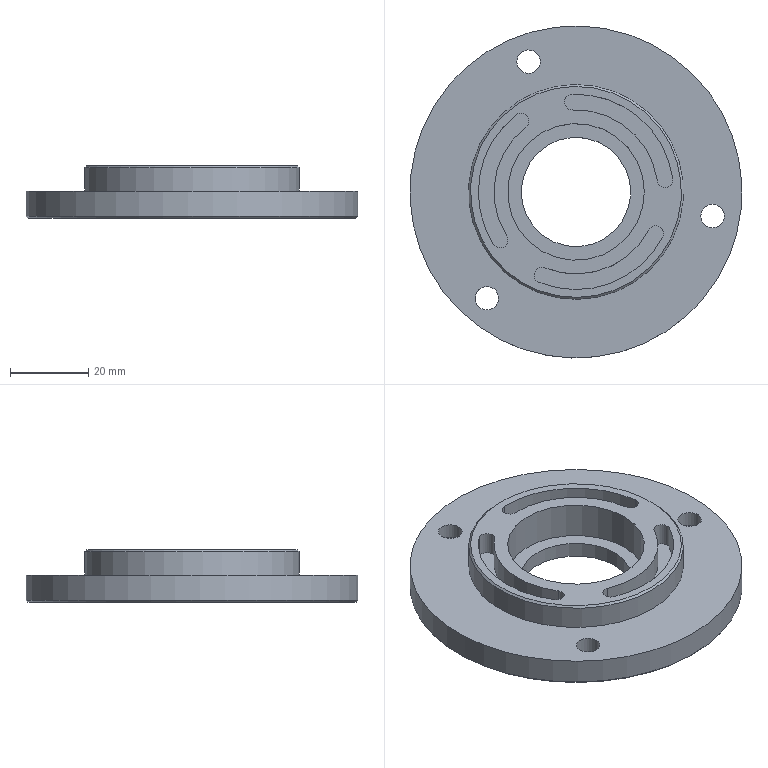Component | NX | CLYB_05_COVERPLATE | 1 solid | 34 faces | volume 39788 mm3 | cylinder 22 | plane 10 | cone 2 | commonest cylinder face diameters 4 x6 6 x3 10 x3 50 x3 42 x3 85 x1 55 x1 28 x1